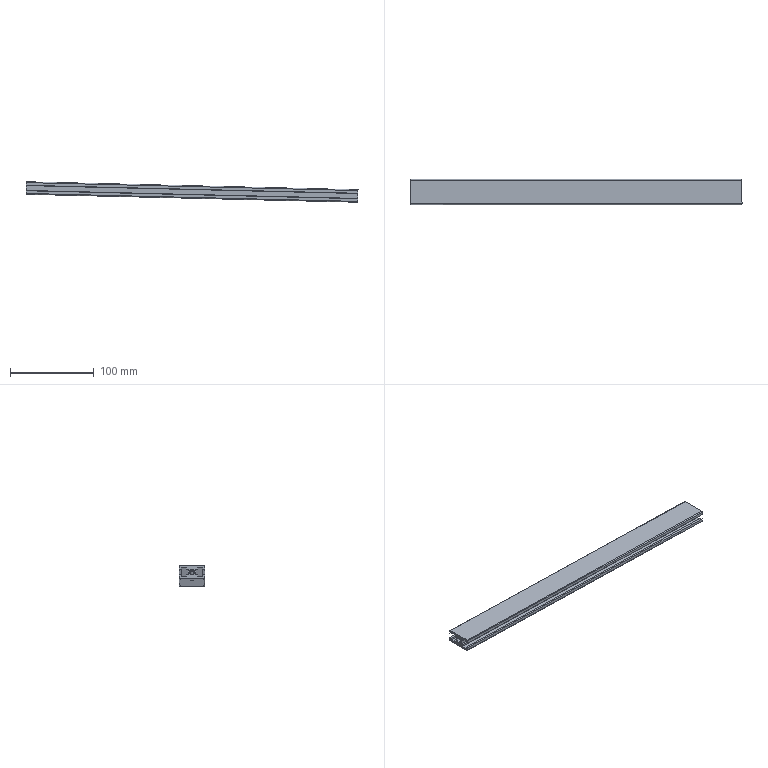Component | SolidWorks | 2012MB0201-1_ASideDoor-1-1_A3002-7 | 1 solid | 58 faces | box 397.25 x 30 x 24.49 mm | volume 96120 mm3 | plane 32 | cylinder 18 | cone 8 | commonest cylinder face diameters 3.3 x8 6 x4 2 x4 5 x2
build123d program:
from build123d import *

# Parameters (mm, degrees)
SKETCH1_2_W                 = 30
SKETCH1_2_H                 = 15
BOSS_EXTRUDE1_DEPTH         = 397
SKETCH2_2_R                 = 2.5
CUT_EXTRUDE1_DEPTH          = 398.354
FILLET1_R                   = 1
M4_TAPPED_HOLE1_D           = 3.3
M4_TAPPED_HOLE1_DEPTH       = 12
M4_TAPPED_HOLE1_CSINK_D     = 4.05
M4_TAPPED_HOLE1_CSINK_ANGLE = 90
M4_TAPPED_HOLE1_TIP         = 0.9914
SKETCH1_R                   = 3
M6_THREADED_END_HOLE1_DEPTH = 13
M6_START                    = -13
SKETCH2_R                   = 3
M6_THREADED_END_HOLE2_DEPTH = 13


with BuildPart() as part:
    # Sketch1_2 → Boss-Extrude1 (new body)
    with BuildSketch(Plane(origin=(0, 0, 0), x_dir=(1, 0, 0), z_dir=(0, 1, 0))):
        Rectangle(SKETCH1_2_W, SKETCH1_2_H)
    extrude(amount=BOSS_EXTRUDE1_DEPTH)

    # Sketch2_2 → Cut-Extrude1 (cut, through all)
    with BuildSketch(Plane.XZ):
        with Locations(Location((0, 0, 0), (0, 0, 270))):
            Circle(SKETCH2_2_R)
        Polygon((15, -3.25), (12.6, -3.25), (12.6, -5.3), (6.6, -5.3), (6.6, -2.926), (4.2, -2.926), (4.2, 2.926), (6.6, 2.926), (6.6, 5.3), (12.6, 5.3), (12.6, 3.25), (15, 3.25), align=None)
        Polygon((-6.6, -2.926), (-4.2, -2.926), (-4.2, 2.926), (-6.6, 2.926), (-6.6, 5.3), (-12.6, 5.3), (-12.6, 3.25), (-15, 3.25), (-15, -3.25), (-12.6, -3.25), (-12.6, -5.3), (-6.6, -5.3), align=None)
    extrude(amount=-CUT_EXTRUDE1_DEPTH, mode=Mode.SUBTRACT)

    # Fillet1
    fillet1_edges = [part.edges().sort_by_distance(p)[0] for p in [
        (15, 198.5, 7.5),
        (-15, 198.5, 7.5),
        (-15, 198.5, -7.5),
        (15, 198.5, -7.5),
    ]]
    fillet(fillet1_edges, radius=FILLET1_R)

    # M4 Tapped Hole1
    with Locations(Plane(origin=(0, 0, -7.5), x_dir=(-1, 0, 0), z_dir=(0, 0, -1))):
        with Locations((0, 70), (0, 86)):
            CounterSinkHole(M4_TAPPED_HOLE1_D / 2, M4_TAPPED_HOLE1_CSINK_D / 2, depth=M4_TAPPED_HOLE1_DEPTH, counter_sink_angle=M4_TAPPED_HOLE1_CSINK_ANGLE)
            with Locations((0, 0, -(M4_TAPPED_HOLE1_DEPTH + M4_TAPPED_HOLE1_TIP / 2))):  # 118° drill point
                Cone(0, M4_TAPPED_HOLE1_D / 2, M4_TAPPED_HOLE1_TIP, mode=Mode.SUBTRACT)

    # Sketch1 → M6 Threaded End Hole1 (cut)
    with BuildSketch(Plane.XZ):
        with Locations(Location((0, 0, 0), (0, 0, 270))):
            Circle(SKETCH1_R)
    extrude(amount=-M6_THREADED_END_HOLE1_DEPTH, mode=Mode.SUBTRACT)

    # Sketch2 → M6 Threaded End Hole2 (cut)
    with BuildSketch(Plane(origin=(0, 397, 0), x_dir=(1, 0, 0), z_dir=(0, 1, 0)).offset(M6_START)):
        with Locations(Location((0, 0, 0), (0, 0, 90))):
            Circle(SKETCH2_R)
    extrude(amount=M6_THREADED_END_HOLE2_DEPTH, mode=Mode.SUBTRACT)


solid = part.part

# Placed as in the assembly
solid = solid.moved(Location((-1249.807, -24.65, -179.612), (0, 1.371, -90)))